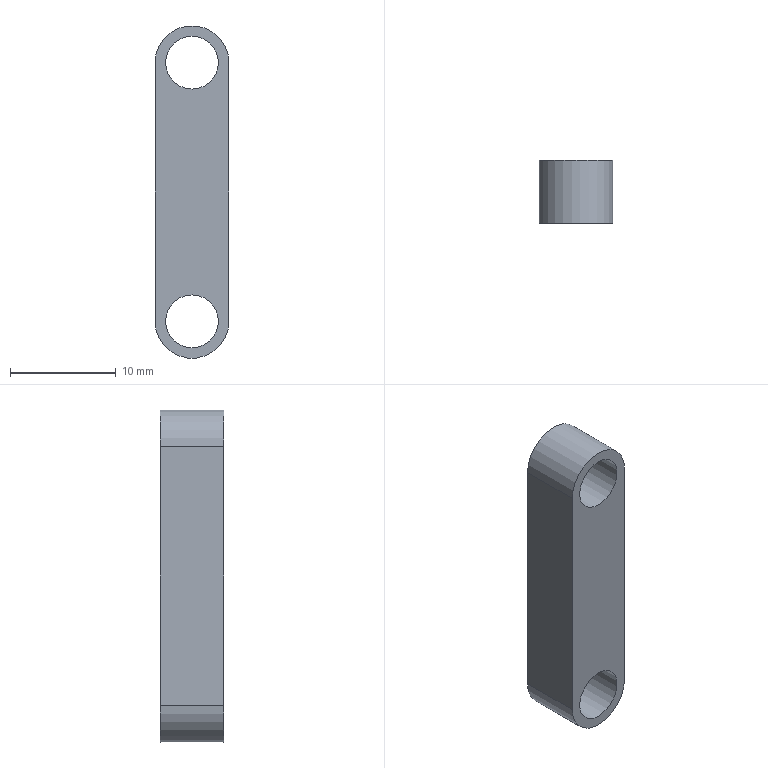Component | NX | LINK | 1 solid | 8 faces | box 7 x 6 x 31.5 mm | volume 1024 mm3 | plane 4 | cylinder 4 | commonest cylinder face diameters 7 x2 5 x2
STEP:
#1=CARTESIAN_POINT('',(0.,0.,0.));
#2=DIRECTION('',(0.,0.,1.));
#3=DIRECTION('',(1.,0.,0.));
#4=AXIS2_PLACEMENT_3D('',#1,#2,#3);
#5=CARTESIAN_POINT('',(9.5,-3.,204.011));
#6=VERTEX_POINT('',#5);
#7=CARTESIAN_POINT('',(9.5,-3.,179.511));
#8=VERTEX_POINT('',#7);
#9=CARTESIAN_POINT('',(9.5,-3.,204.011));
#10=DIRECTION('',(0.,0.,-1.));
#11=VECTOR('',#10,1.);
#12=LINE('',#9,#11);
#13=CARTESIAN_POINT('',(9.5,3.,204.011));
#14=DIRECTION('',(-1.,0.,-0.));
#15=DIRECTION('',(-0.,0.,1.));
#16=AXIS2_PLACEMENT_3D('',#13,#14,#15);
#17=PLANE('',#16);
#18=CARTESIAN_POINT('',(0.,-6.));
#19=DIRECTION('',(-1.,0.));
#20=VECTOR('',#19,1.);
#21=LINE('',#18,#20);
#22=(GEOMETRIC_REPRESENTATION_CONTEXT(2)PARAMETRIC_REPRESENTATION_CONTEXT()REPRESENTATION_CONTEXT('',''));
#23=DEFINITIONAL_REPRESENTATION('',(#21),#22);
#24=PCURVE('',#17,#23);
#25=CARTESIAN_POINT('',(6.,-3.,179.511));
#26=DIRECTION('',(0.,1.,0.));
#27=DIRECTION('',(1.,0.,0.));
#28=AXIS2_PLACEMENT_3D('',#25,#26,#27);
#29=PLANE('',#28);
#30=CARTESIAN_POINT('',(3.5,-24.5));
#31=DIRECTION('',(0.,1.));
#32=VECTOR('',#31,1.);
#33=LINE('',#30,#32);
#34=(GEOMETRIC_REPRESENTATION_CONTEXT(2)PARAMETRIC_REPRESENTATION_CONTEXT()REPRESENTATION_CONTEXT('',''));
#35=DEFINITIONAL_REPRESENTATION('',(#33),#34);
#36=PCURVE('',#29,#35);
#37=SURFACE_CURVE('',#12,(#24,#36),.PCURVE_S1.);
#38=EDGE_CURVE('',#6,#8,#37,.T.);
#39=ORIENTED_EDGE('',*,*,#38,.T.);
#40=CARTESIAN_POINT('',(9.5,3.,179.511));
#41=VERTEX_POINT('',#40);
#42=CARTESIAN_POINT('',(9.5,3.,179.511));
#43=DIRECTION('',(0.,-1.,0.));
#44=VECTOR('',#43,1.);
#45=LINE('',#42,#44);
#46=CARTESIAN_POINT('',(-24.5,0.));
#47=DIRECTION('',(0.,-1.));
#48=VECTOR('',#47,1.);
#49=LINE('',#46,#48);
#50=(GEOMETRIC_REPRESENTATION_CONTEXT(2)PARAMETRIC_REPRESENTATION_CONTEXT()REPRESENTATION_CONTEXT('',''));
#51=DEFINITIONAL_REPRESENTATION('',(#49),#50);
#52=PCURVE('',#17,#51);
#53=CARTESIAN_POINT('',(6.,3.,179.511));
#54=DIRECTION('',(0.,-1.,0.));
#55=DIRECTION('',(-1.,0.,0.));
#56=AXIS2_PLACEMENT_3D('',#53,#54,#55);
#57=CYLINDRICAL_SURFACE('',#56,3.5);
#58=CARTESIAN_POINT('',(3.142,0.));
#59=DIRECTION('',(0.,1.));
#60=VECTOR('',#59,1.);
#61=LINE('',#58,#60);
#62=(GEOMETRIC_REPRESENTATION_CONTEXT(2)PARAMETRIC_REPRESENTATION_CONTEXT()REPRESENTATION_CONTEXT('',''));
#63=DEFINITIONAL_REPRESENTATION('',(#61),#62);
#64=PCURVE('',#57,#63);
#65=SURFACE_CURVE('',#45,(#52,#64),.PCURVE_S1.);
#66=EDGE_CURVE('',#41,#8,#65,.T.);
#67=ORIENTED_EDGE('',*,*,#66,.F.);
#68=CARTESIAN_POINT('',(9.5,3.,204.011));
#69=VERTEX_POINT('',#68);
#70=CARTESIAN_POINT('',(9.5,3.,204.011));
#71=DIRECTION('',(0.,0.,-1.));
#72=VECTOR('',#71,1.);
#73=LINE('',#70,#72);
#74=CARTESIAN_POINT('',(0.,0.));
#75=DIRECTION('',(-1.,0.));
#76=VECTOR('',#75,1.);
#77=LINE('',#74,#76);
#78=(GEOMETRIC_REPRESENTATION_CONTEXT(2)PARAMETRIC_REPRESENTATION_CONTEXT()REPRESENTATION_CONTEXT('',''));
#79=DEFINITIONAL_REPRESENTATION('',(#77),#78);
#80=PCURVE('',#17,#79);
#81=CARTESIAN_POINT('',(6.,3.,179.511));
#82=DIRECTION('',(0.,1.,0.));
#83=DIRECTION('',(1.,0.,0.));
#84=AXIS2_PLACEMENT_3D('',#81,#82,#83);
#85=PLANE('',#84);
#86=CARTESIAN_POINT('',(3.5,-24.5));
#87=DIRECTION('',(0.,1.));
#88=VECTOR('',#87,1.);
#89=LINE('',#86,#88);
#90=(GEOMETRIC_REPRESENTATION_CONTEXT(2)PARAMETRIC_REPRESENTATION_CONTEXT()REPRESENTATION_CONTEXT('',''));
#91=DEFINITIONAL_REPRESENTATION('',(#89),#90);
#92=PCURVE('',#85,#91);
#93=SURFACE_CURVE('',#73,(#80,#92),.PCURVE_S1.);
#94=EDGE_CURVE('',#69,#41,#93,.T.);
#95=ORIENTED_EDGE('',*,*,#94,.F.);
#96=CARTESIAN_POINT('',(9.5,3.,204.011));
#97=DIRECTION('',(0.,-1.,0.));
#98=VECTOR('',#97,1.);
#99=LINE('',#96,#98);
#100=CARTESIAN_POINT('',(0.,0.));
#101=DIRECTION('',(0.,-1.));
#102=VECTOR('',#101,1.);
#103=LINE('',#100,#102);
#104=(GEOMETRIC_REPRESENTATION_CONTEXT(2)PARAMETRIC_REPRESENTATION_CONTEXT()REPRESENTATION_CONTEXT('',''));
#105=DEFINITIONAL_REPRESENTATION('',(#103),#104);
#106=PCURVE('',#17,#105);
#107=CARTESIAN_POINT('',(6.,3.,204.011));
#108=DIRECTION('',(0.,-1.,0.));
#109=DIRECTION('',(-1.,0.,0.));
#110=AXIS2_PLACEMENT_3D('',#107,#108,#109);
#111=CYLINDRICAL_SURFACE('',#110,3.5);
#112=CARTESIAN_POINT('',(3.142,0.));
#113=DIRECTION('',(0.,1.));
#114=VECTOR('',#113,1.);
#115=LINE('',#112,#114);
#116=(GEOMETRIC_REPRESENTATION_CONTEXT(2)PARAMETRIC_REPRESENTATION_CONTEXT()REPRESENTATION_CONTEXT('',''));
#117=DEFINITIONAL_REPRESENTATION('',(#115),#116);
#118=PCURVE('',#111,#117);
#119=SURFACE_CURVE('',#99,(#106,#118),.PCURVE_S1.);
#120=EDGE_CURVE('',#69,#6,#119,.T.);
#121=ORIENTED_EDGE('',*,*,#120,.T.);
#122=EDGE_LOOP('',(#39,#67,#95,#121));
#123=FACE_BOUND('',#122,.T.);
#124=ADVANCED_FACE('',(#123),#17,.F.);
#125=CARTESIAN_POINT('',(2.5,-3.,179.511));
#126=VERTEX_POINT('',#125);
#127=CARTESIAN_POINT('',(6.,-3.,179.511));
#128=DIRECTION('',(0.,1.,0.));
#129=DIRECTION('',(0.,0.,-1.));
#130=AXIS2_PLACEMENT_3D('',#127,#128,#129);
#131=CIRCLE('',#130,3.5);
#132=CARTESIAN_POINT('',(7.854,6.));
#133=DIRECTION('',(-1.,0.));
#134=VECTOR('',#133,1.);
#135=LINE('',#132,#134);
#136=(GEOMETRIC_REPRESENTATION_CONTEXT(2)PARAMETRIC_REPRESENTATION_CONTEXT()REPRESENTATION_CONTEXT('',''));
#137=DEFINITIONAL_REPRESENTATION('',(#135),#136);
#138=PCURVE('',#57,#137);
#139=CARTESIAN_POINT('',(0.,0.));
#140=DIRECTION('',(0.,1.));
#141=AXIS2_PLACEMENT_2D('',#139,#140);
#142=CIRCLE('',#141,3.5);
#143=(GEOMETRIC_REPRESENTATION_CONTEXT(2)PARAMETRIC_REPRESENTATION_CONTEXT()REPRESENTATION_CONTEXT('',''));
#144=DEFINITIONAL_REPRESENTATION('',(#142),#143);
#145=PCURVE('',#29,#144);
#146=SURFACE_CURVE('',#131,(#138,#145),.PCURVE_S1.);
#147=EDGE_CURVE('',#8,#126,#146,.T.);
#148=ORIENTED_EDGE('',*,*,#147,.T.);
#149=CARTESIAN_POINT('',(2.5,3.,179.511));
#150=VERTEX_POINT('',#149);
#151=CARTESIAN_POINT('',(2.5,3.,179.511));
#152=DIRECTION('',(0.,-1.,0.));
#153=VECTOR('',#152,1.);
#154=LINE('',#151,#153);
#155=CARTESIAN_POINT('',(0.,0.));
#156=DIRECTION('',(0.,1.));
#157=VECTOR('',#156,1.);
#158=LINE('',#155,#157);
#159=(GEOMETRIC_REPRESENTATION_CONTEXT(2)PARAMETRIC_REPRESENTATION_CONTEXT()REPRESENTATION_CONTEXT('',''));
#160=DEFINITIONAL_REPRESENTATION('',(#158),#159);
#161=PCURVE('',#57,#160);
#162=CARTESIAN_POINT('',(2.5,3.,179.511));
#163=DIRECTION('',(1.,0.,-0.));
#164=DIRECTION('',(-0.,0.,-1.));
#165=AXIS2_PLACEMENT_3D('',#162,#163,#164);
#166=PLANE('',#165);
#167=CARTESIAN_POINT('',(0.,0.));
#168=DIRECTION('',(0.,-1.));
#169=VECTOR('',#168,1.);
#170=LINE('',#167,#169);
#171=(GEOMETRIC_REPRESENTATION_CONTEXT(2)PARAMETRIC_REPRESENTATION_CONTEXT()REPRESENTATION_CONTEXT('',''));
#172=DEFINITIONAL_REPRESENTATION('',(#170),#171);
#173=PCURVE('',#166,#172);
#174=SURFACE_CURVE('',#154,(#161,#173),.PCURVE_S1.);
#175=EDGE_CURVE('',#150,#126,#174,.T.);
#176=ORIENTED_EDGE('',*,*,#175,.F.);
#177=CARTESIAN_POINT('',(6.,3.,179.511));
#178=DIRECTION('',(0.,1.,0.));
#179=DIRECTION('',(0.,0.,-1.));
#180=AXIS2_PLACEMENT_3D('',#177,#178,#179);
#181=CIRCLE('',#180,3.5);
#182=CARTESIAN_POINT('',(7.854,0.));
#183=DIRECTION('',(-1.,0.));
#184=VECTOR('',#183,1.);
#185=LINE('',#182,#184);
#186=(GEOMETRIC_REPRESENTATION_CONTEXT(2)PARAMETRIC_REPRESENTATION_CONTEXT()REPRESENTATION_CONTEXT('',''));
#187=DEFINITIONAL_REPRESENTATION('',(#185),#186);
#188=PCURVE('',#57,#187);
#189=CARTESIAN_POINT('',(0.,0.));
#190=DIRECTION('',(0.,1.));
#191=AXIS2_PLACEMENT_2D('',#189,#190);
#192=CIRCLE('',#191,3.5);
#193=(GEOMETRIC_REPRESENTATION_CONTEXT(2)PARAMETRIC_REPRESENTATION_CONTEXT()REPRESENTATION_CONTEXT('',''));
#194=DEFINITIONAL_REPRESENTATION('',(#192),#193);
#195=PCURVE('',#85,#194);
#196=SURFACE_CURVE('',#181,(#188,#195),.PCURVE_S1.);
#197=EDGE_CURVE('',#41,#150,#196,.T.);
#198=ORIENTED_EDGE('',*,*,#197,.F.);
#199=ORIENTED_EDGE('',*,*,#66,.T.);
#200=EDGE_LOOP('',(#148,#176,#198,#199));
#201=FACE_BOUND('',#200,.T.);
#202=ADVANCED_FACE('',(#201),#57,.T.);
#203=CARTESIAN_POINT('',(2.5,-3.,204.011));
#204=VERTEX_POINT('',#203);
#205=CARTESIAN_POINT('',(2.5,-3.,179.511));
#206=DIRECTION('',(0.,0.,1.));
#207=VECTOR('',#206,1.);
#208=LINE('',#205,#207);
#209=CARTESIAN_POINT('',(0.,-6.));
#210=DIRECTION('',(-1.,0.));
#211=VECTOR('',#210,1.);
#212=LINE('',#209,#211);
#213=(GEOMETRIC_REPRESENTATION_CONTEXT(2)PARAMETRIC_REPRESENTATION_CONTEXT()REPRESENTATION_CONTEXT('',''));
#214=DEFINITIONAL_REPRESENTATION('',(#212),#213);
#215=PCURVE('',#166,#214);
#216=CARTESIAN_POINT('',(-3.5,0.));
#217=DIRECTION('',(0.,-1.));
#218=VECTOR('',#217,1.);
#219=LINE('',#216,#218);
#220=(GEOMETRIC_REPRESENTATION_CONTEXT(2)PARAMETRIC_REPRESENTATION_CONTEXT()REPRESENTATION_CONTEXT('',''));
#221=DEFINITIONAL_REPRESENTATION('',(#219),#220);
#222=PCURVE('',#29,#221);
#223=SURFACE_CURVE('',#208,(#215,#222),.PCURVE_S1.);
#224=EDGE_CURVE('',#126,#204,#223,.T.);
#225=ORIENTED_EDGE('',*,*,#224,.T.);
#226=CARTESIAN_POINT('',(2.5,3.,204.011));
#227=VERTEX_POINT('',#226);
#228=CARTESIAN_POINT('',(2.5,3.,204.011));
#229=DIRECTION('',(0.,-1.,0.));
#230=VECTOR('',#229,1.);
#231=LINE('',#228,#230);
#232=CARTESIAN_POINT('',(-24.5,0.));
#233=DIRECTION('',(0.,-1.));
#234=VECTOR('',#233,1.);
#235=LINE('',#232,#234);
#236=(GEOMETRIC_REPRESENTATION_CONTEXT(2)PARAMETRIC_REPRESENTATION_CONTEXT()REPRESENTATION_CONTEXT('',''));
#237=DEFINITIONAL_REPRESENTATION('',(#235),#236);
#238=PCURVE('',#166,#237);
#239=CARTESIAN_POINT('',(6.283,0.));
#240=DIRECTION('',(0.,1.));
#241=VECTOR('',#240,1.);
#242=LINE('',#239,#241);
#243=(GEOMETRIC_REPRESENTATION_CONTEXT(2)PARAMETRIC_REPRESENTATION_CONTEXT()REPRESENTATION_CONTEXT('',''));
#244=DEFINITIONAL_REPRESENTATION('',(#242),#243);
#245=PCURVE('',#111,#244);
#246=SURFACE_CURVE('',#231,(#238,#245),.PCURVE_S1.);
#247=EDGE_CURVE('',#227,#204,#246,.T.);
#248=ORIENTED_EDGE('',*,*,#247,.F.);
#249=CARTESIAN_POINT('',(2.5,3.,179.511));
#250=DIRECTION('',(0.,0.,1.));
#251=VECTOR('',#250,1.);
#252=LINE('',#249,#251);
#253=CARTESIAN_POINT('',(0.,0.));
#254=DIRECTION('',(-1.,0.));
#255=VECTOR('',#254,1.);
#256=LINE('',#253,#255);
#257=(GEOMETRIC_REPRESENTATION_CONTEXT(2)PARAMETRIC_REPRESENTATION_CONTEXT()REPRESENTATION_CONTEXT('',''));
#258=DEFINITIONAL_REPRESENTATION('',(#256),#257);
#259=PCURVE('',#166,#258);
#260=CARTESIAN_POINT('',(-3.5,0.));
#261=DIRECTION('',(0.,-1.));
#262=VECTOR('',#261,1.);
#263=LINE('',#260,#262);
#264=(GEOMETRIC_REPRESENTATION_CONTEXT(2)PARAMETRIC_REPRESENTATION_CONTEXT()REPRESENTATION_CONTEXT('',''));
#265=DEFINITIONAL_REPRESENTATION('',(#263),#264);
#266=PCURVE('',#85,#265);
#267=SURFACE_CURVE('',#252,(#259,#266),.PCURVE_S1.);
#268=EDGE_CURVE('',#150,#227,#267,.T.);
#269=ORIENTED_EDGE('',*,*,#268,.F.);
#270=ORIENTED_EDGE('',*,*,#175,.T.);
#271=EDGE_LOOP('',(#225,#248,#269,#270));
#272=FACE_BOUND('',#271,.T.);
#273=ADVANCED_FACE('',(#272),#166,.F.);
#274=CARTESIAN_POINT('',(6.,-3.,204.011));
#275=DIRECTION('',(0.,1.,0.));
#276=DIRECTION('',(0.,0.,-1.));
#277=AXIS2_PLACEMENT_3D('',#274,#275,#276);
#278=CIRCLE('',#277,3.5);
#279=CARTESIAN_POINT('',(7.854,6.));
#280=DIRECTION('',(-1.,0.));
#281=VECTOR('',#280,1.);
#282=LINE('',#279,#281);
#283=(GEOMETRIC_REPRESENTATION_CONTEXT(2)PARAMETRIC_REPRESENTATION_CONTEXT()REPRESENTATION_CONTEXT('',''));
#284=DEFINITIONAL_REPRESENTATION('',(#282),#283);
#285=PCURVE('',#111,#284);
#286=CARTESIAN_POINT('',(0.,-24.5));
#287=DIRECTION('',(0.,1.));
#288=AXIS2_PLACEMENT_2D('',#286,#287);
#289=CIRCLE('',#288,3.5);
#290=(GEOMETRIC_REPRESENTATION_CONTEXT(2)PARAMETRIC_REPRESENTATION_CONTEXT()REPRESENTATION_CONTEXT('',''));
#291=DEFINITIONAL_REPRESENTATION('',(#289),#290);
#292=PCURVE('',#29,#291);
#293=SURFACE_CURVE('',#278,(#285,#292),.PCURVE_S1.);
#294=EDGE_CURVE('',#204,#6,#293,.T.);
#295=ORIENTED_EDGE('',*,*,#294,.T.);
#296=ORIENTED_EDGE('',*,*,#120,.F.);
#297=CARTESIAN_POINT('',(6.,3.,204.011));
#298=DIRECTION('',(0.,1.,0.));
#299=DIRECTION('',(0.,0.,-1.));
#300=AXIS2_PLACEMENT_3D('',#297,#298,#299);
#301=CIRCLE('',#300,3.5);
#302=CARTESIAN_POINT('',(7.854,0.));
#303=DIRECTION('',(-1.,0.));
#304=VECTOR('',#303,1.);
#305=LINE('',#302,#304);
#306=(GEOMETRIC_REPRESENTATION_CONTEXT(2)PARAMETRIC_REPRESENTATION_CONTEXT()REPRESENTATION_CONTEXT('',''));
#307=DEFINITIONAL_REPRESENTATION('',(#305),#306);
#308=PCURVE('',#111,#307);
#309=CARTESIAN_POINT('',(0.,-24.5));
#310=DIRECTION('',(0.,1.));
#311=AXIS2_PLACEMENT_2D('',#309,#310);
#312=CIRCLE('',#311,3.5);
#313=(GEOMETRIC_REPRESENTATION_CONTEXT(2)PARAMETRIC_REPRESENTATION_CONTEXT()REPRESENTATION_CONTEXT('',''));
#314=DEFINITIONAL_REPRESENTATION('',(#312),#313);
#315=PCURVE('',#85,#314);
#316=SURFACE_CURVE('',#301,(#308,#315),.PCURVE_S1.);
#317=EDGE_CURVE('',#227,#69,#316,.T.);
#318=ORIENTED_EDGE('',*,*,#317,.F.);
#319=ORIENTED_EDGE('',*,*,#247,.T.);
#320=EDGE_LOOP('',(#295,#296,#318,#319));
#321=FACE_BOUND('',#320,.T.);
#322=ADVANCED_FACE('',(#321),#111,.T.);
#323=CARTESIAN_POINT('',(6.,3.,177.011));
#324=VERTEX_POINT('',#323);
#325=CARTESIAN_POINT('',(6.,3.,179.511));
#326=DIRECTION('',(0.,-1.,0.));
#327=DIRECTION('',(0.,0.,-1.));
#328=AXIS2_PLACEMENT_3D('',#325,#326,#327);
#329=CIRCLE('',#328,2.5);
#330=CARTESIAN_POINT('',(0.,2.5));
#331=CARTESIAN_POINT('',(4.33,2.5));
#332=CARTESIAN_POINT('',(2.165,-1.25));
#333=CARTESIAN_POINT('',(0.,-5.));
#334=CARTESIAN_POINT('',(-2.165,-1.25));
#335=CARTESIAN_POINT('',(-4.33,2.5));
#336=CARTESIAN_POINT('',(0.,2.5));
#337=(BOUNDED_CURVE()B_SPLINE_CURVE(2,(#330,#331,#332,#333,#334,#335,#336),.UNSPECIFIED.,.T.,.F.)B_SPLINE_CURVE_WITH_KNOTS((1,2,2,2,2,1),(-2.094,0.,2.094,4.189,6.283,8.378),.UNSPECIFIED.)CURVE()GEOMETRIC_REPRESENTATION_ITEM()RATIONAL_B_SPLINE_CURVE((1.,0.5,1.,0.5,1.,0.5,1.))REPRESENTATION_ITEM(''));
#338=(GEOMETRIC_REPRESENTATION_CONTEXT(2)PARAMETRIC_REPRESENTATION_CONTEXT()REPRESENTATION_CONTEXT('',''));
#339=DEFINITIONAL_REPRESENTATION('',(#337),#338);
#340=PCURVE('',#85,#339);
#341=CARTESIAN_POINT('',(6.,3.,179.511));
#342=DIRECTION('',(0.,-1.,0.));
#343=DIRECTION('',(-1.,0.,0.));
#344=AXIS2_PLACEMENT_3D('',#341,#342,#343);
#345=CYLINDRICAL_SURFACE('',#344,2.5);
#346=CARTESIAN_POINT('',(1.571,0.));
#347=DIRECTION('',(1.,0.));
#348=VECTOR('',#347,1.);
#349=LINE('',#346,#348);
#350=(GEOMETRIC_REPRESENTATION_CONTEXT(2)PARAMETRIC_REPRESENTATION_CONTEXT()REPRESENTATION_CONTEXT('',''));
#351=DEFINITIONAL_REPRESENTATION('',(#349),#350);
#352=PCURVE('',#345,#351);
#353=SURFACE_CURVE('',#329,(#340,#352),.PCURVE_S1.);
#354=EDGE_CURVE('',#324,#324,#353,.T.);
#355=ORIENTED_EDGE('',*,*,#354,.T.);
#356=EDGE_LOOP('',(#355));
#357=FACE_BOUND('',#356,.T.);
#358=CARTESIAN_POINT('',(6.,3.,201.511));
#359=VERTEX_POINT('',#358);
#360=CARTESIAN_POINT('',(6.,3.,204.011));
#361=DIRECTION('',(0.,-1.,0.));
#362=DIRECTION('',(0.,0.,-1.));
#363=AXIS2_PLACEMENT_3D('',#360,#361,#362);
#364=CIRCLE('',#363,2.5);
#365=CARTESIAN_POINT('',(0.,-22.));
#366=CARTESIAN_POINT('',(4.33,-22.));
#367=CARTESIAN_POINT('',(2.165,-25.75));
#368=CARTESIAN_POINT('',(0.,-29.5));
#369=CARTESIAN_POINT('',(-2.165,-25.75));
#370=CARTESIAN_POINT('',(-4.33,-22.));
#371=CARTESIAN_POINT('',(0.,-22.));
#372=(BOUNDED_CURVE()B_SPLINE_CURVE(2,(#365,#366,#367,#368,#369,#370,#371),.UNSPECIFIED.,.T.,.F.)B_SPLINE_CURVE_WITH_KNOTS((1,2,2,2,2,1),(-2.094,0.,2.094,4.189,6.283,8.378),.UNSPECIFIED.)CURVE()GEOMETRIC_REPRESENTATION_ITEM()RATIONAL_B_SPLINE_CURVE((1.,0.5,1.,0.5,1.,0.5,1.))REPRESENTATION_ITEM(''));
#373=(GEOMETRIC_REPRESENTATION_CONTEXT(2)PARAMETRIC_REPRESENTATION_CONTEXT()REPRESENTATION_CONTEXT('',''));
#374=DEFINITIONAL_REPRESENTATION('',(#372),#373);
#375=PCURVE('',#85,#374);
#376=CARTESIAN_POINT('',(6.,3.,204.011));
#377=DIRECTION('',(0.,-1.,0.));
#378=DIRECTION('',(-1.,0.,0.));
#379=AXIS2_PLACEMENT_3D('',#376,#377,#378);
#380=CYLINDRICAL_SURFACE('',#379,2.5);
#381=CARTESIAN_POINT('',(1.571,0.));
#382=DIRECTION('',(1.,0.));
#383=VECTOR('',#382,1.);
#384=LINE('',#381,#383);
#385=(GEOMETRIC_REPRESENTATION_CONTEXT(2)PARAMETRIC_REPRESENTATION_CONTEXT()REPRESENTATION_CONTEXT('',''));
#386=DEFINITIONAL_REPRESENTATION('',(#384),#385);
#387=PCURVE('',#380,#386);
#388=SURFACE_CURVE('',#364,(#375,#387),.PCURVE_S1.);
#389=EDGE_CURVE('',#359,#359,#388,.T.);
#390=ORIENTED_EDGE('',*,*,#389,.T.);
#391=EDGE_LOOP('',(#390));
#392=FACE_BOUND('',#391,.T.);
#393=ORIENTED_EDGE('',*,*,#94,.T.);
#394=ORIENTED_EDGE('',*,*,#197,.T.);
#395=ORIENTED_EDGE('',*,*,#268,.T.);
#396=ORIENTED_EDGE('',*,*,#317,.T.);
#397=EDGE_LOOP('',(#393,#394,#395,#396));
#398=FACE_BOUND('',#397,.T.);
#399=ADVANCED_FACE('',(#357,#392,#398),#85,.T.);
#400=CARTESIAN_POINT('',(6.,-3.,177.011));
#401=VERTEX_POINT('',#400);
#402=CARTESIAN_POINT('',(6.,-3.,179.511));
#403=DIRECTION('',(0.,-1.,0.));
#404=DIRECTION('',(0.,0.,-1.));
#405=AXIS2_PLACEMENT_3D('',#402,#403,#404);
#406=CIRCLE('',#405,2.5);
#407=CARTESIAN_POINT('',(0.,2.5));
#408=CARTESIAN_POINT('',(4.33,2.5));
#409=CARTESIAN_POINT('',(2.165,-1.25));
#410=CARTESIAN_POINT('',(0.,-5.));
#411=CARTESIAN_POINT('',(-2.165,-1.25));
#412=CARTESIAN_POINT('',(-4.33,2.5));
#413=CARTESIAN_POINT('',(0.,2.5));
#414=(BOUNDED_CURVE()B_SPLINE_CURVE(2,(#407,#408,#409,#410,#411,#412,#413),.UNSPECIFIED.,.T.,.F.)B_SPLINE_CURVE_WITH_KNOTS((1,2,2,2,2,1),(-2.094,0.,2.094,4.189,6.283,8.378),.UNSPECIFIED.)CURVE()GEOMETRIC_REPRESENTATION_ITEM()RATIONAL_B_SPLINE_CURVE((1.,0.5,1.,0.5,1.,0.5,1.))REPRESENTATION_ITEM(''));
#415=(GEOMETRIC_REPRESENTATION_CONTEXT(2)PARAMETRIC_REPRESENTATION_CONTEXT()REPRESENTATION_CONTEXT('',''));
#416=DEFINITIONAL_REPRESENTATION('',(#414),#415);
#417=PCURVE('',#29,#416);
#418=CARTESIAN_POINT('',(1.571,6.));
#419=DIRECTION('',(1.,0.));
#420=VECTOR('',#419,1.);
#421=LINE('',#418,#420);
#422=(GEOMETRIC_REPRESENTATION_CONTEXT(2)PARAMETRIC_REPRESENTATION_CONTEXT()REPRESENTATION_CONTEXT('',''));
#423=DEFINITIONAL_REPRESENTATION('',(#421),#422);
#424=PCURVE('',#345,#423);
#425=SURFACE_CURVE('',#406,(#417,#424),.PCURVE_S1.);
#426=EDGE_CURVE('',#401,#401,#425,.T.);
#427=ORIENTED_EDGE('',*,*,#426,.F.);
#428=EDGE_LOOP('',(#427));
#429=FACE_BOUND('',#428,.T.);
#430=CARTESIAN_POINT('',(6.,-3.,201.511));
#431=VERTEX_POINT('',#430);
#432=CARTESIAN_POINT('',(6.,-3.,204.011));
#433=DIRECTION('',(0.,-1.,0.));
#434=DIRECTION('',(0.,0.,-1.));
#435=AXIS2_PLACEMENT_3D('',#432,#433,#434);
#436=CIRCLE('',#435,2.5);
#437=CARTESIAN_POINT('',(0.,-22.));
#438=CARTESIAN_POINT('',(4.33,-22.));
#439=CARTESIAN_POINT('',(2.165,-25.75));
#440=CARTESIAN_POINT('',(0.,-29.5));
#441=CARTESIAN_POINT('',(-2.165,-25.75));
#442=CARTESIAN_POINT('',(-4.33,-22.));
#443=CARTESIAN_POINT('',(0.,-22.));
#444=(BOUNDED_CURVE()B_SPLINE_CURVE(2,(#437,#438,#439,#440,#441,#442,#443),.UNSPECIFIED.,.T.,.F.)B_SPLINE_CURVE_WITH_KNOTS((1,2,2,2,2,1),(-2.094,0.,2.094,4.189,6.283,8.378),.UNSPECIFIED.)CURVE()GEOMETRIC_REPRESENTATION_ITEM()RATIONAL_B_SPLINE_CURVE((1.,0.5,1.,0.5,1.,0.5,1.))REPRESENTATION_ITEM(''));
#445=(GEOMETRIC_REPRESENTATION_CONTEXT(2)PARAMETRIC_REPRESENTATION_CONTEXT()REPRESENTATION_CONTEXT('',''));
#446=DEFINITIONAL_REPRESENTATION('',(#444),#445);
#447=PCURVE('',#29,#446);
#448=CARTESIAN_POINT('',(1.571,6.));
#449=DIRECTION('',(1.,0.));
#450=VECTOR('',#449,1.);
#451=LINE('',#448,#450);
#452=(GEOMETRIC_REPRESENTATION_CONTEXT(2)PARAMETRIC_REPRESENTATION_CONTEXT()REPRESENTATION_CONTEXT('',''));
#453=DEFINITIONAL_REPRESENTATION('',(#451),#452);
#454=PCURVE('',#380,#453);
#455=SURFACE_CURVE('',#436,(#447,#454),.PCURVE_S1.);
#456=EDGE_CURVE('',#431,#431,#455,.T.);
#457=ORIENTED_EDGE('',*,*,#456,.F.);
#458=EDGE_LOOP('',(#457));
#459=FACE_BOUND('',#458,.T.);
#460=ORIENTED_EDGE('',*,*,#38,.F.);
#461=ORIENTED_EDGE('',*,*,#294,.F.);
#462=ORIENTED_EDGE('',*,*,#224,.F.);
#463=ORIENTED_EDGE('',*,*,#147,.F.);
#464=EDGE_LOOP('',(#460,#461,#462,#463));
#465=FACE_BOUND('',#464,.T.);
#466=ADVANCED_FACE('',(#429,#459,#465),#29,.F.);
#467=ORIENTED_EDGE('',*,*,#389,.T.);
#468=CARTESIAN_POINT('',(6.,3.,201.511));
#469=CARTESIAN_POINT('',(6.,-3.,201.511));
#470=B_SPLINE_CURVE_WITH_KNOTS('',1,(#468,#469),.UNSPECIFIED.,.F.,.F.,(2,2),(0.,6.),.PIECEWISE_BEZIER_KNOTS.);
#471=CARTESIAN_POINT('',(7.854,0.));
#472=DIRECTION('',(0.,1.));
#473=VECTOR('',#472,1.);
#474=LINE('',#471,#473);
#475=(GEOMETRIC_REPRESENTATION_CONTEXT(2)PARAMETRIC_REPRESENTATION_CONTEXT()REPRESENTATION_CONTEXT('',''));
#476=DEFINITIONAL_REPRESENTATION('',(#474),#475);
#477=PCURVE('',#380,#476);
#478=CARTESIAN_POINT('',(1.571,0.));
#479=DIRECTION('',(0.,1.));
#480=VECTOR('',#479,1.);
#481=LINE('',#478,#480);
#482=(GEOMETRIC_REPRESENTATION_CONTEXT(2)PARAMETRIC_REPRESENTATION_CONTEXT()REPRESENTATION_CONTEXT('',''));
#483=DEFINITIONAL_REPRESENTATION('',(#481),#482);
#484=PCURVE('',#380,#483);
#485=SEAM_CURVE('',#470,(#477,#484),.PCURVE_S1.);
#486=EDGE_CURVE('',#359,#431,#485,.T.);
#487=ORIENTED_EDGE('',*,*,#486,.T.);
#488=ORIENTED_EDGE('',*,*,#456,.F.);
#489=ORIENTED_EDGE('',*,*,#486,.F.);
#490=EDGE_LOOP('',(#467,#487,#488,#489));
#491=FACE_BOUND('',#490,.F.);
#492=ADVANCED_FACE('',(#491),#380,.F.);
#493=ORIENTED_EDGE('',*,*,#354,.T.);
#494=CARTESIAN_POINT('',(6.,3.,177.011));
#495=CARTESIAN_POINT('',(6.,-3.,177.011));
#496=B_SPLINE_CURVE_WITH_KNOTS('',1,(#494,#495),.UNSPECIFIED.,.F.,.F.,(2,2),(0.,6.),.PIECEWISE_BEZIER_KNOTS.);
#497=CARTESIAN_POINT('',(7.854,0.));
#498=DIRECTION('',(0.,1.));
#499=VECTOR('',#498,1.);
#500=LINE('',#497,#499);
#501=(GEOMETRIC_REPRESENTATION_CONTEXT(2)PARAMETRIC_REPRESENTATION_CONTEXT()REPRESENTATION_CONTEXT('',''));
#502=DEFINITIONAL_REPRESENTATION('',(#500),#501);
#503=PCURVE('',#345,#502);
#504=CARTESIAN_POINT('',(1.571,0.));
#505=DIRECTION('',(0.,1.));
#506=VECTOR('',#505,1.);
#507=LINE('',#504,#506);
#508=(GEOMETRIC_REPRESENTATION_CONTEXT(2)PARAMETRIC_REPRESENTATION_CONTEXT()REPRESENTATION_CONTEXT('',''));
#509=DEFINITIONAL_REPRESENTATION('',(#507),#508);
#510=PCURVE('',#345,#509);
#511=SEAM_CURVE('',#496,(#503,#510),.PCURVE_S1.);
#512=EDGE_CURVE('',#324,#401,#511,.T.);
#513=ORIENTED_EDGE('',*,*,#512,.T.);
#514=ORIENTED_EDGE('',*,*,#426,.F.);
#515=ORIENTED_EDGE('',*,*,#512,.F.);
#516=EDGE_LOOP('',(#493,#513,#514,#515));
#517=FACE_BOUND('',#516,.F.);
#518=ADVANCED_FACE('',(#517),#345,.F.);
#519=CLOSED_SHELL('',(#124,#202,#273,#322,#399,#466,#492,#518));
#520=MANIFOLD_SOLID_BREP('',#519);
#521=(LENGTH_UNIT()NAMED_UNIT(*)SI_UNIT(.MILLI.,.METRE.));
#522=UNCERTAINTY_MEASURE_WITH_UNIT(LENGTH_MEASURE(0.000002),#521,'','');
#523=(NAMED_UNIT(*)PLANE_ANGLE_UNIT()SI_UNIT($,.RADIAN.));
#524=(NAMED_UNIT(*)SI_UNIT($,.STERADIAN.)SOLID_ANGLE_UNIT());
#525=(GEOMETRIC_REPRESENTATION_CONTEXT(3)GLOBAL_UNCERTAINTY_ASSIGNED_CONTEXT((#522))GLOBAL_UNIT_ASSIGNED_CONTEXT((#521,#523,#524))REPRESENTATION_CONTEXT('',''));
#526=ADVANCED_BREP_SHAPE_REPRESENTATION('',(#4,#520),#525);